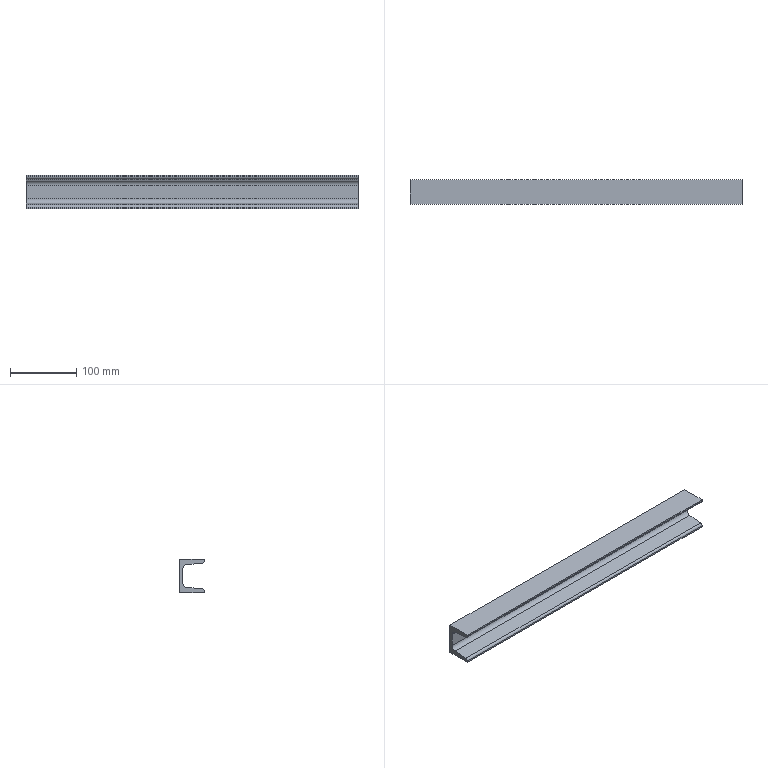Component | SolidWorks | 002FrameBaseAssembly-1_hot-rolled steel channel gb-10 | 1 solid | 14 faces | box 500 x 37 x 50 mm | volume 346226 mm3 | plane 10 | cylinder 4 | commonest cylinder face diameters 14 x2 7 x2
build123d program:
from build123d import *

# Parameters (mm, degrees)
BASE_DEPTH = 500
FILLET1_R  = 7
FILLET2_R  = 3.5


with BuildPart() as part:
    # Sketch1 → Base (new body)
    with BuildSketch(Plane(origin=(0, 0, -28.211), x_dir=(0, 0, 1), z_dir=(1, 0, 0))):
        Polygon((28.211, -25), (28.211, 25), (65.211, 25), (65.211, 19.625), (32.711, 16.375), (32.711, -16.375), (65.211, -19.625), (65.211, -25), align=None)
    extrude(amount=BASE_DEPTH)

    # Fillet1
    fillet1_edges = [part.edges().sort_by_distance(p)[0] for p in [
        (250, -16.375, 4.5),
        (250, 16.375, 4.5),
    ]]
    fillet(fillet1_edges, radius=FILLET1_R)

    # Fillet2
    fillet2_edges = [part.edges().sort_by_distance(p)[0] for p in [
        (250, 19.625, 37),
        (250, -19.625, 37),
    ]]
    fillet(fillet2_edges, radius=FILLET2_R)


solid = part.part

# Placed as in the assembly
solid = solid.moved(Location((-120, 37, -40), (90, 0, 0)))
STEP:
#1=CARTESIAN_POINT('',(-4.724,0.1241,-2.335));
#2=VERTEX_POINT('',#1);
#3=CARTESIAN_POINT('',(-4.724,1.031,-2.244));
#4=VERTEX_POINT('',#3);
#5=CARTESIAN_POINT('',(-4.724,1.28,-2.219));
#6=DIRECTION('',(0.,0.995,0.0995));
#7=VECTOR('',#6,39.37);
#8=LINE('',#5,#7);
#9=EDGE_CURVE('',#2,#4,#8,.T.);
#10=ORIENTED_EDGE('',*,*,#9,.F.);
#11=CARTESIAN_POINT('',(14.961,0.1241,-2.335));
#12=VERTEX_POINT('',#11);
#13=CARTESIAN_POINT('',(-4.724,0.1241,-2.335));
#14=DIRECTION('',(1.,-0.,0.));
#15=VECTOR('',#14,39.37);
#16=LINE('',#13,#15);
#17=EDGE_CURVE('',#2,#12,#16,.T.);
#18=ORIENTED_EDGE('',*,*,#17,.T.);
#19=CARTESIAN_POINT('',(14.961,1.031,-2.244));
#20=VERTEX_POINT('',#19);
#21=CARTESIAN_POINT('',(14.961,1.28,-2.219));
#22=DIRECTION('',(0.,0.995,0.0995));
#23=VECTOR('',#22,39.37);
#24=LINE('',#21,#23);
#25=EDGE_CURVE('',#12,#20,#24,.T.);
#26=ORIENTED_EDGE('',*,*,#25,.T.);
#27=CARTESIAN_POINT('',(-4.724,1.031,-2.244));
#28=DIRECTION('',(-1.,0.,0.));
#29=VECTOR('',#28,39.37);
#30=LINE('',#27,#29);
#31=EDGE_CURVE('',#20,#4,#30,.T.);
#32=ORIENTED_EDGE('',*,*,#31,.T.);
#33=EDGE_LOOP('',(#10,#18,#26,#32));
#34=FACE_OUTER_BOUND('',#33,.T.);
#35=CARTESIAN_POINT('',(-4.724,1.28,-2.219));
#36=DIRECTION('',(0.,0.0995,-0.995));
#37=DIRECTION('',(-0.,-0.995,-0.0995));
#38=AXIS2_PLACEMENT_3D('',#35,#36,#37);
#39=PLANE('',#38);
#40=ADVANCED_FACE('',(#34),#39,.F.);
#41=CARTESIAN_POINT('',(14.961,1.28,-1.97));
#42=VERTEX_POINT('',#41);
#43=CARTESIAN_POINT('',(14.961,1.28,-1.18));
#44=VERTEX_POINT('',#43);
#45=CARTESIAN_POINT('',(14.961,1.28,-0.9301));
#46=DIRECTION('',(0.,0.,1.));
#47=VECTOR('',#46,39.37);
#48=LINE('',#45,#47);
#49=EDGE_CURVE('',#42,#44,#48,.T.);
#50=ORIENTED_EDGE('',*,*,#49,.T.);
#51=CARTESIAN_POINT('',(-4.724,1.28,-1.18));
#52=VERTEX_POINT('',#51);
#53=CARTESIAN_POINT('',(-4.724,1.28,-1.18));
#54=DIRECTION('',(-1.,0.,0.));
#55=VECTOR('',#54,39.37);
#56=LINE('',#53,#55);
#57=EDGE_CURVE('',#44,#52,#56,.T.);
#58=ORIENTED_EDGE('',*,*,#57,.T.);
#59=CARTESIAN_POINT('',(-4.724,1.28,-1.97));
#60=VERTEX_POINT('',#59);
#61=CARTESIAN_POINT('',(-4.724,1.28,-0.9301));
#62=DIRECTION('',(0.,0.,1.));
#63=VECTOR('',#62,39.37);
#64=LINE('',#61,#63);
#65=EDGE_CURVE('',#60,#52,#64,.T.);
#66=ORIENTED_EDGE('',*,*,#65,.F.);
#67=CARTESIAN_POINT('',(14.961,1.28,-1.97));
#68=DIRECTION('',(1.,-0.,0.));
#69=VECTOR('',#68,39.37);
#70=LINE('',#67,#69);
#71=EDGE_CURVE('',#60,#42,#70,.T.);
#72=ORIENTED_EDGE('',*,*,#71,.T.);
#73=EDGE_LOOP('',(#50,#58,#66,#72));
#74=FACE_OUTER_BOUND('',#73,.T.);
#75=CARTESIAN_POINT('',(-4.724,1.28,-0.9301));
#76=DIRECTION('',(0.,1.,-0.));
#77=DIRECTION('',(1.,-0.,0.));
#78=AXIS2_PLACEMENT_3D('',#75,#76,#77);
#79=PLANE('',#78);
#80=ADVANCED_FACE('',(#74),#79,.F.);
#81=CARTESIAN_POINT('',(14.961,1.031,-0.9053));
#82=VERTEX_POINT('',#81);
#83=CARTESIAN_POINT('',(14.961,0.1241,-0.8146));
#84=VERTEX_POINT('',#83);
#85=CARTESIAN_POINT('',(14.961,1.28,-0.9301));
#86=DIRECTION('',(-0.,-0.995,0.0995));
#87=VECTOR('',#86,39.37);
#88=LINE('',#85,#87);
#89=EDGE_CURVE('',#82,#84,#88,.T.);
#90=ORIENTED_EDGE('',*,*,#89,.T.);
#91=CARTESIAN_POINT('',(-4.724,0.1241,-0.8146));
#92=VERTEX_POINT('',#91);
#93=CARTESIAN_POINT('',(-4.724,0.1241,-0.8146));
#94=DIRECTION('',(-1.,0.,0.));
#95=VECTOR('',#94,39.37);
#96=LINE('',#93,#95);
#97=EDGE_CURVE('',#84,#92,#96,.T.);
#98=ORIENTED_EDGE('',*,*,#97,.T.);
#99=CARTESIAN_POINT('',(-4.724,1.031,-0.9053));
#100=VERTEX_POINT('',#99);
#101=CARTESIAN_POINT('',(-4.724,1.28,-0.9301));
#102=DIRECTION('',(-0.,-0.995,0.0995));
#103=VECTOR('',#102,39.37);
#104=LINE('',#101,#103);
#105=EDGE_CURVE('',#100,#92,#104,.T.);
#106=ORIENTED_EDGE('',*,*,#105,.F.);
#107=CARTESIAN_POINT('',(14.961,1.031,-0.9053));
#108=DIRECTION('',(1.,-0.,0.));
#109=VECTOR('',#108,39.37);
#110=LINE('',#107,#109);
#111=EDGE_CURVE('',#100,#82,#110,.T.);
#112=ORIENTED_EDGE('',*,*,#111,.T.);
#113=EDGE_LOOP('',(#90,#98,#106,#112));
#114=FACE_OUTER_BOUND('',#113,.T.);
#115=CARTESIAN_POINT('',(-4.724,1.28,-0.9301));
#116=DIRECTION('',(0.,0.0995,0.995));
#117=DIRECTION('',(0.,0.995,-0.0995));
#118=AXIS2_PLACEMENT_3D('',#115,#116,#117);
#119=PLANE('',#118);
#120=ADVANCED_FACE('',(#114),#119,.F.);
#121=CARTESIAN_POINT('',(-4.724,0.,-0.6775));
#122=VERTEX_POINT('',#121);
#123=CARTESIAN_POINT('',(-4.724,0.,-0.5906));
#124=VERTEX_POINT('',#123);
#125=CARTESIAN_POINT('',(-4.724,0.,-0.8022));
#126=DIRECTION('',(0.,0.,1.));
#127=VECTOR('',#126,39.37);
#128=LINE('',#125,#127);
#129=EDGE_CURVE('',#122,#124,#128,.T.);
#130=ORIENTED_EDGE('',*,*,#129,.F.);
#131=CARTESIAN_POINT('',(14.961,-0.,-0.6775));
#132=VERTEX_POINT('',#131);
#133=CARTESIAN_POINT('',(-4.724,0.,-0.6775));
#134=DIRECTION('',(1.,-0.,0.));
#135=VECTOR('',#134,39.37);
#136=LINE('',#133,#135);
#137=EDGE_CURVE('',#122,#132,#136,.T.);
#138=ORIENTED_EDGE('',*,*,#137,.T.);
#139=CARTESIAN_POINT('',(14.961,-0.,-0.5906));
#140=VERTEX_POINT('',#139);
#141=CARTESIAN_POINT('',(14.961,-0.,-0.8022));
#142=DIRECTION('',(0.,0.,1.));
#143=VECTOR('',#142,39.37);
#144=LINE('',#141,#143);
#145=EDGE_CURVE('',#132,#140,#144,.T.);
#146=ORIENTED_EDGE('',*,*,#145,.T.);
#147=CARTESIAN_POINT('',(-4.724,0.,-0.5906));
#148=DIRECTION('',(1.,-0.,0.));
#149=VECTOR('',#148,39.37);
#150=LINE('',#147,#149);
#151=EDGE_CURVE('',#124,#140,#150,.T.);
#152=ORIENTED_EDGE('',*,*,#151,.F.);
#153=EDGE_LOOP('',(#130,#138,#146,#152));
#154=FACE_OUTER_BOUND('',#153,.T.);
#155=CARTESIAN_POINT('',(-4.724,0.,-0.8022));
#156=DIRECTION('',(0.,1.,-0.));
#157=DIRECTION('',(1.,-0.,0.));
#158=AXIS2_PLACEMENT_3D('',#155,#156,#157);
#159=PLANE('',#158);
#160=ADVANCED_FACE('',(#154),#159,.F.);
#161=CARTESIAN_POINT('',(14.961,1.457,-0.5906));
#162=VERTEX_POINT('',#161);
#163=CARTESIAN_POINT('',(14.961,1.457,-0.5906));
#164=DIRECTION('',(0.,1.,-0.));
#165=VECTOR('',#164,39.37);
#166=LINE('',#163,#165);
#167=EDGE_CURVE('',#140,#162,#166,.T.);
#168=ORIENTED_EDGE('',*,*,#167,.T.);
#169=CARTESIAN_POINT('',(-4.724,1.457,-0.5906));
#170=VERTEX_POINT('',#169);
#171=CARTESIAN_POINT('',(-4.724,1.457,-0.5906));
#172=DIRECTION('',(1.,-0.,0.));
#173=VECTOR('',#172,39.37);
#174=LINE('',#171,#173);
#175=EDGE_CURVE('',#170,#162,#174,.T.);
#176=ORIENTED_EDGE('',*,*,#175,.F.);
#177=CARTESIAN_POINT('',(-4.724,1.457,-0.5906));
#178=DIRECTION('',(0.,1.,-0.));
#179=VECTOR('',#178,39.37);
#180=LINE('',#177,#179);
#181=EDGE_CURVE('',#124,#170,#180,.T.);
#182=ORIENTED_EDGE('',*,*,#181,.F.);
#183=ORIENTED_EDGE('',*,*,#151,.T.);
#184=EDGE_LOOP('',(#168,#176,#182,#183));
#185=FACE_OUTER_BOUND('',#184,.T.);
#186=CARTESIAN_POINT('',(-4.724,1.457,-0.5906));
#187=DIRECTION('',(-0.,-0.,-1.));
#188=DIRECTION('',(-0.,-1.,0.));
#189=AXIS2_PLACEMENT_3D('',#186,#187,#188);
#190=PLANE('',#189);
#191=ADVANCED_FACE('',(#185),#190,.F.);
#192=CARTESIAN_POINT('',(14.961,1.457,-2.559));
#193=VERTEX_POINT('',#192);
#194=CARTESIAN_POINT('',(14.961,1.457,-2.559));
#195=DIRECTION('',(0.,0.,-1.));
#196=VECTOR('',#195,39.37);
#197=LINE('',#194,#196);
#198=EDGE_CURVE('',#162,#193,#197,.T.);
#199=ORIENTED_EDGE('',*,*,#198,.T.);
#200=CARTESIAN_POINT('',(-4.724,1.457,-2.559));
#201=VERTEX_POINT('',#200);
#202=CARTESIAN_POINT('',(-4.724,1.457,-2.559));
#203=DIRECTION('',(1.,-0.,0.));
#204=VECTOR('',#203,39.37);
#205=LINE('',#202,#204);
#206=EDGE_CURVE('',#201,#193,#205,.T.);
#207=ORIENTED_EDGE('',*,*,#206,.F.);
#208=CARTESIAN_POINT('',(-4.724,1.457,-2.559));
#209=DIRECTION('',(0.,0.,-1.));
#210=VECTOR('',#209,39.37);
#211=LINE('',#208,#210);
#212=EDGE_CURVE('',#170,#201,#211,.T.);
#213=ORIENTED_EDGE('',*,*,#212,.F.);
#214=ORIENTED_EDGE('',*,*,#175,.T.);
#215=EDGE_LOOP('',(#199,#207,#213,#214));
#216=FACE_OUTER_BOUND('',#215,.T.);
#217=CARTESIAN_POINT('',(-4.724,1.457,-2.559));
#218=DIRECTION('',(-0.,-1.,-0.));
#219=DIRECTION('',(-0.,-0.,1.));
#220=AXIS2_PLACEMENT_3D('',#217,#218,#219);
#221=PLANE('',#220);
#222=ADVANCED_FACE('',(#216),#221,.F.);
#223=CARTESIAN_POINT('',(14.961,-0.,-2.559));
#224=VERTEX_POINT('',#223);
#225=CARTESIAN_POINT('',(14.961,1.457,-2.559));
#226=DIRECTION('',(-0.,-1.,0.));
#227=VECTOR('',#226,39.37);
#228=LINE('',#225,#227);
#229=EDGE_CURVE('',#193,#224,#228,.T.);
#230=ORIENTED_EDGE('',*,*,#229,.T.);
#231=CARTESIAN_POINT('',(-4.724,0.,-2.559));
#232=VERTEX_POINT('',#231);
#233=CARTESIAN_POINT('',(-4.724,0.,-2.559));
#234=DIRECTION('',(1.,-0.,0.));
#235=VECTOR('',#234,39.37);
#236=LINE('',#233,#235);
#237=EDGE_CURVE('',#232,#224,#236,.T.);
#238=ORIENTED_EDGE('',*,*,#237,.F.);
#239=CARTESIAN_POINT('',(-4.724,1.457,-2.559));
#240=DIRECTION('',(-0.,-1.,0.));
#241=VECTOR('',#240,39.37);
#242=LINE('',#239,#241);
#243=EDGE_CURVE('',#201,#232,#242,.T.);
#244=ORIENTED_EDGE('',*,*,#243,.F.);
#245=ORIENTED_EDGE('',*,*,#206,.T.);
#246=EDGE_LOOP('',(#230,#238,#244,#245));
#247=FACE_OUTER_BOUND('',#246,.T.);
#248=CARTESIAN_POINT('',(-4.724,1.457,-2.559));
#249=DIRECTION('',(0.,0.,1.));
#250=DIRECTION('',(0.,1.,-0.));
#251=AXIS2_PLACEMENT_3D('',#248,#249,#250);
#252=PLANE('',#251);
#253=ADVANCED_FACE('',(#247),#252,.F.);
#254=CARTESIAN_POINT('',(14.961,-0.,-2.472));
#255=VERTEX_POINT('',#254);
#256=CARTESIAN_POINT('',(14.961,-0.,-2.347));
#257=DIRECTION('',(0.,0.,1.));
#258=VECTOR('',#257,39.37);
#259=LINE('',#256,#258);
#260=EDGE_CURVE('',#224,#255,#259,.T.);
#261=ORIENTED_EDGE('',*,*,#260,.T.);
#262=CARTESIAN_POINT('',(-4.724,0.,-2.472));
#263=VERTEX_POINT('',#262);
#264=CARTESIAN_POINT('',(-4.724,0.,-2.472));
#265=DIRECTION('',(-1.,0.,0.));
#266=VECTOR('',#265,39.37);
#267=LINE('',#264,#266);
#268=EDGE_CURVE('',#255,#263,#267,.T.);
#269=ORIENTED_EDGE('',*,*,#268,.T.);
#270=CARTESIAN_POINT('',(-4.724,0.,-2.347));
#271=DIRECTION('',(0.,0.,1.));
#272=VECTOR('',#271,39.37);
#273=LINE('',#270,#272);
#274=EDGE_CURVE('',#232,#263,#273,.T.);
#275=ORIENTED_EDGE('',*,*,#274,.F.);
#276=ORIENTED_EDGE('',*,*,#237,.T.);
#277=EDGE_LOOP('',(#261,#269,#275,#276));
#278=FACE_OUTER_BOUND('',#277,.T.);
#279=CARTESIAN_POINT('',(-4.724,0.,-2.347));
#280=DIRECTION('',(0.,1.,-0.));
#281=DIRECTION('',(1.,-0.,0.));
#282=AXIS2_PLACEMENT_3D('',#279,#280,#281);
#283=PLANE('',#282);
#284=ADVANCED_FACE('',(#278),#283,.F.);
#285=ORIENTED_EDGE('',*,*,#105,.T.);
#286=CARTESIAN_POINT('',(-4.724,0.1378,-0.6775));
#287=DIRECTION('',(-1.,0.,0.));
#288=DIRECTION('',(0.,1.,0.));
#289=AXIS2_PLACEMENT_3D('',#286,#287,#288);
#290=CIRCLE('',#289,0.1378);
#291=EDGE_CURVE('',#92,#122,#290,.T.);
#292=ORIENTED_EDGE('',*,*,#291,.T.);
#293=ORIENTED_EDGE('',*,*,#129,.T.);
#294=ORIENTED_EDGE('',*,*,#181,.T.);
#295=ORIENTED_EDGE('',*,*,#212,.T.);
#296=ORIENTED_EDGE('',*,*,#243,.T.);
#297=ORIENTED_EDGE('',*,*,#274,.T.);
#298=CARTESIAN_POINT('',(-4.724,0.1378,-2.472));
#299=DIRECTION('',(-1.,0.,0.));
#300=DIRECTION('',(0.,1.,0.));
#301=AXIS2_PLACEMENT_3D('',#298,#299,#300);
#302=CIRCLE('',#301,0.1378);
#303=EDGE_CURVE('',#263,#2,#302,.T.);
#304=ORIENTED_EDGE('',*,*,#303,.T.);
#305=ORIENTED_EDGE('',*,*,#9,.T.);
#306=CARTESIAN_POINT('',(-4.724,1.004,-1.97));
#307=DIRECTION('',(1.,-0.,0.));
#308=DIRECTION('',(0.,1.,0.));
#309=AXIS2_PLACEMENT_3D('',#306,#307,#308);
#310=CIRCLE('',#309,0.2756);
#311=EDGE_CURVE('',#4,#60,#310,.T.);
#312=ORIENTED_EDGE('',*,*,#311,.T.);
#313=ORIENTED_EDGE('',*,*,#65,.T.);
#314=CARTESIAN_POINT('',(-4.724,1.004,-1.18));
#315=DIRECTION('',(1.,-0.,0.));
#316=DIRECTION('',(0.,1.,0.));
#317=AXIS2_PLACEMENT_3D('',#314,#315,#316);
#318=CIRCLE('',#317,0.2756);
#319=EDGE_CURVE('',#52,#100,#318,.T.);
#320=ORIENTED_EDGE('',*,*,#319,.T.);
#321=EDGE_LOOP('',(#285,#292,#293,#294,#295,#296,#297,#304,#305,#312,#313,#320));
#322=FACE_OUTER_BOUND('',#321,.T.);
#323=CARTESIAN_POINT('',(-4.724,1.457,-2.202));
#324=DIRECTION('',(-1.,0.,0.));
#325=DIRECTION('',(0.,1.,-0.));
#326=AXIS2_PLACEMENT_3D('',#323,#324,#325);
#327=PLANE('',#326);
#328=ADVANCED_FACE('',(#322),#327,.T.);
#329=ORIENTED_EDGE('',*,*,#145,.F.);
#330=CARTESIAN_POINT('',(14.961,0.1378,-0.6775));
#331=DIRECTION('',(1.,-0.,0.));
#332=DIRECTION('',(0.,1.,0.));
#333=AXIS2_PLACEMENT_3D('',#330,#331,#332);
#334=CIRCLE('',#333,0.1378);
#335=EDGE_CURVE('',#132,#84,#334,.T.);
#336=ORIENTED_EDGE('',*,*,#335,.T.);
#337=ORIENTED_EDGE('',*,*,#89,.F.);
#338=CARTESIAN_POINT('',(14.961,1.004,-1.18));
#339=DIRECTION('',(-1.,0.,0.));
#340=DIRECTION('',(0.,1.,0.));
#341=AXIS2_PLACEMENT_3D('',#338,#339,#340);
#342=CIRCLE('',#341,0.2756);
#343=EDGE_CURVE('',#82,#44,#342,.T.);
#344=ORIENTED_EDGE('',*,*,#343,.T.);
#345=ORIENTED_EDGE('',*,*,#49,.F.);
#346=CARTESIAN_POINT('',(14.961,1.004,-1.97));
#347=DIRECTION('',(-1.,0.,0.));
#348=DIRECTION('',(0.,1.,0.));
#349=AXIS2_PLACEMENT_3D('',#346,#347,#348);
#350=CIRCLE('',#349,0.2756);
#351=EDGE_CURVE('',#42,#20,#350,.T.);
#352=ORIENTED_EDGE('',*,*,#351,.T.);
#353=ORIENTED_EDGE('',*,*,#25,.F.);
#354=CARTESIAN_POINT('',(14.961,0.1378,-2.472));
#355=DIRECTION('',(1.,-0.,0.));
#356=DIRECTION('',(0.,1.,0.));
#357=AXIS2_PLACEMENT_3D('',#354,#355,#356);
#358=CIRCLE('',#357,0.1378);
#359=EDGE_CURVE('',#12,#255,#358,.T.);
#360=ORIENTED_EDGE('',*,*,#359,.T.);
#361=ORIENTED_EDGE('',*,*,#260,.F.);
#362=ORIENTED_EDGE('',*,*,#229,.F.);
#363=ORIENTED_EDGE('',*,*,#198,.F.);
#364=ORIENTED_EDGE('',*,*,#167,.F.);
#365=EDGE_LOOP('',(#329,#336,#337,#344,#345,#352,#353,#360,#361,#362,#363,#364));
#366=FACE_OUTER_BOUND('',#365,.T.);
#367=CARTESIAN_POINT('',(14.961,1.457,-2.202));
#368=DIRECTION('',(-1.,0.,0.));
#369=DIRECTION('',(0.,1.,-0.));
#370=AXIS2_PLACEMENT_3D('',#367,#368,#369);
#371=PLANE('',#370);
#372=ADVANCED_FACE('',(#366),#371,.F.);
#373=ORIENTED_EDGE('',*,*,#319,.F.);
#374=ORIENTED_EDGE('',*,*,#57,.F.);
#375=ORIENTED_EDGE('',*,*,#343,.F.);
#376=ORIENTED_EDGE('',*,*,#111,.F.);
#377=EDGE_LOOP('',(#373,#374,#375,#376));
#378=FACE_OUTER_BOUND('',#377,.T.);
#379=CARTESIAN_POINT('',(-4.724,1.004,-1.18));
#380=DIRECTION('',(-1.,0.,0.));
#381=DIRECTION('',(0.,1.,0.));
#382=AXIS2_PLACEMENT_3D('',#379,#380,#381);
#383=CYLINDRICAL_SURFACE('',#382,0.2756);
#384=ADVANCED_FACE('',(#378),#383,.F.);
#385=ORIENTED_EDGE('',*,*,#311,.F.);
#386=ORIENTED_EDGE('',*,*,#31,.F.);
#387=ORIENTED_EDGE('',*,*,#351,.F.);
#388=ORIENTED_EDGE('',*,*,#71,.F.);
#389=EDGE_LOOP('',(#385,#386,#387,#388));
#390=FACE_OUTER_BOUND('',#389,.T.);
#391=CARTESIAN_POINT('',(-4.724,1.004,-1.97));
#392=DIRECTION('',(-1.,0.,0.));
#393=DIRECTION('',(0.,1.,0.));
#394=AXIS2_PLACEMENT_3D('',#391,#392,#393);
#395=CYLINDRICAL_SURFACE('',#394,0.2756);
#396=ADVANCED_FACE('',(#390),#395,.F.);
#397=ORIENTED_EDGE('',*,*,#291,.F.);
#398=ORIENTED_EDGE('',*,*,#97,.F.);
#399=ORIENTED_EDGE('',*,*,#335,.F.);
#400=ORIENTED_EDGE('',*,*,#137,.F.);
#401=EDGE_LOOP('',(#397,#398,#399,#400));
#402=FACE_OUTER_BOUND('',#401,.T.);
#403=CARTESIAN_POINT('',(-4.724,0.1378,-0.6775));
#404=DIRECTION('',(1.,-0.,0.));
#405=DIRECTION('',(0.,-1.,0.));
#406=AXIS2_PLACEMENT_3D('',#403,#404,#405);
#407=CYLINDRICAL_SURFACE('',#406,0.1378);
#408=ADVANCED_FACE('',(#402),#407,.T.);
#409=ORIENTED_EDGE('',*,*,#303,.F.);
#410=ORIENTED_EDGE('',*,*,#268,.F.);
#411=ORIENTED_EDGE('',*,*,#359,.F.);
#412=ORIENTED_EDGE('',*,*,#17,.F.);
#413=EDGE_LOOP('',(#409,#410,#411,#412));
#414=FACE_OUTER_BOUND('',#413,.T.);
#415=CARTESIAN_POINT('',(-4.724,0.1378,-2.472));
#416=DIRECTION('',(1.,-0.,0.));
#417=DIRECTION('',(0.,-1.,0.));
#418=AXIS2_PLACEMENT_3D('',#415,#416,#417);
#419=CYLINDRICAL_SURFACE('',#418,0.1378);
#420=ADVANCED_FACE('',(#414),#419,.T.);
#421=CLOSED_SHELL('',(#40,#80,#120,#160,#191,#222,#253,#284,#328,#372,#384,#396,#408,#420));
#422=MANIFOLD_SOLID_BREP('',#421);
#423=CARTESIAN_POINT('',(0.,0.,0.));
#424=DIRECTION('',(0.,0.,1.));
#425=DIRECTION('',(1.,0.,0.));
#426=AXIS2_PLACEMENT_3D('',#423,#424,#425);
#427=(LENGTH_UNIT()NAMED_UNIT(*)SI_UNIT($,.METRE.));
#428=LENGTH_MEASURE_WITH_UNIT(LENGTH_MEASURE(0.0254),#427);
#429=DIMENSIONAL_EXPONENTS(1.,0.,0.,0.,0.,0.,0.);
#430=(CONVERSION_BASED_UNIT('',#428)LENGTH_UNIT()NAMED_UNIT(#429));
#431=UNCERTAINTY_MEASURE_WITH_UNIT(LENGTH_MEASURE(0.00001),#430,'','');
#432=(NAMED_UNIT(*)PLANE_ANGLE_UNIT()SI_UNIT($,.RADIAN.));
#433=(NAMED_UNIT(*)SI_UNIT($,.STERADIAN.)SOLID_ANGLE_UNIT());
#434=(GEOMETRIC_REPRESENTATION_CONTEXT(3)GLOBAL_UNCERTAINTY_ASSIGNED_CONTEXT((#431))GLOBAL_UNIT_ASSIGNED_CONTEXT((#430,#432,#433))REPRESENTATION_CONTEXT('',''));
#435=ADVANCED_BREP_SHAPE_REPRESENTATION('',(#422,#426),#434);
#436=COLOUR_RGB('',0.7922,0.8196,0.9333);
#437=FILL_AREA_STYLE_COLOUR('',#436);
#438=FILL_AREA_STYLE('',(#437));
#439=SURFACE_STYLE_FILL_AREA(#438);
#440=SURFACE_SIDE_STYLE('',(#439));
#441=SURFACE_STYLE_USAGE(.BOTH.,#440);
#442=PRESENTATION_STYLE_ASSIGNMENT((#441));
#443=STYLED_ITEM('',(#442),#422);
#444=PRESENTATION_LAYER_ASSIGNMENT('','',(#443));
#445=(LENGTH_UNIT()NAMED_UNIT(*)SI_UNIT($,.METRE.));
#446=LENGTH_MEASURE_WITH_UNIT(LENGTH_MEASURE(0.0254),#445);
#447=DIMENSIONAL_EXPONENTS(1.,0.,0.,0.,0.,0.,0.);
#448=(CONVERSION_BASED_UNIT('',#446)LENGTH_UNIT()NAMED_UNIT(#447));
#449=UNCERTAINTY_MEASURE_WITH_UNIT(LENGTH_MEASURE(0.00001),#448,'','');
#450=(NAMED_UNIT(*)PLANE_ANGLE_UNIT()SI_UNIT($,.RADIAN.));
#451=(NAMED_UNIT(*)SI_UNIT($,.STERADIAN.)SOLID_ANGLE_UNIT());
#452=(GEOMETRIC_REPRESENTATION_CONTEXT(3)GLOBAL_UNCERTAINTY_ASSIGNED_CONTEXT((#449))GLOBAL_UNIT_ASSIGNED_CONTEXT((#448,#450,#451))REPRESENTATION_CONTEXT('',''));
#453=MECHANICAL_DESIGN_GEOMETRIC_PRESENTATION_REPRESENTATION('',(#443),#452);